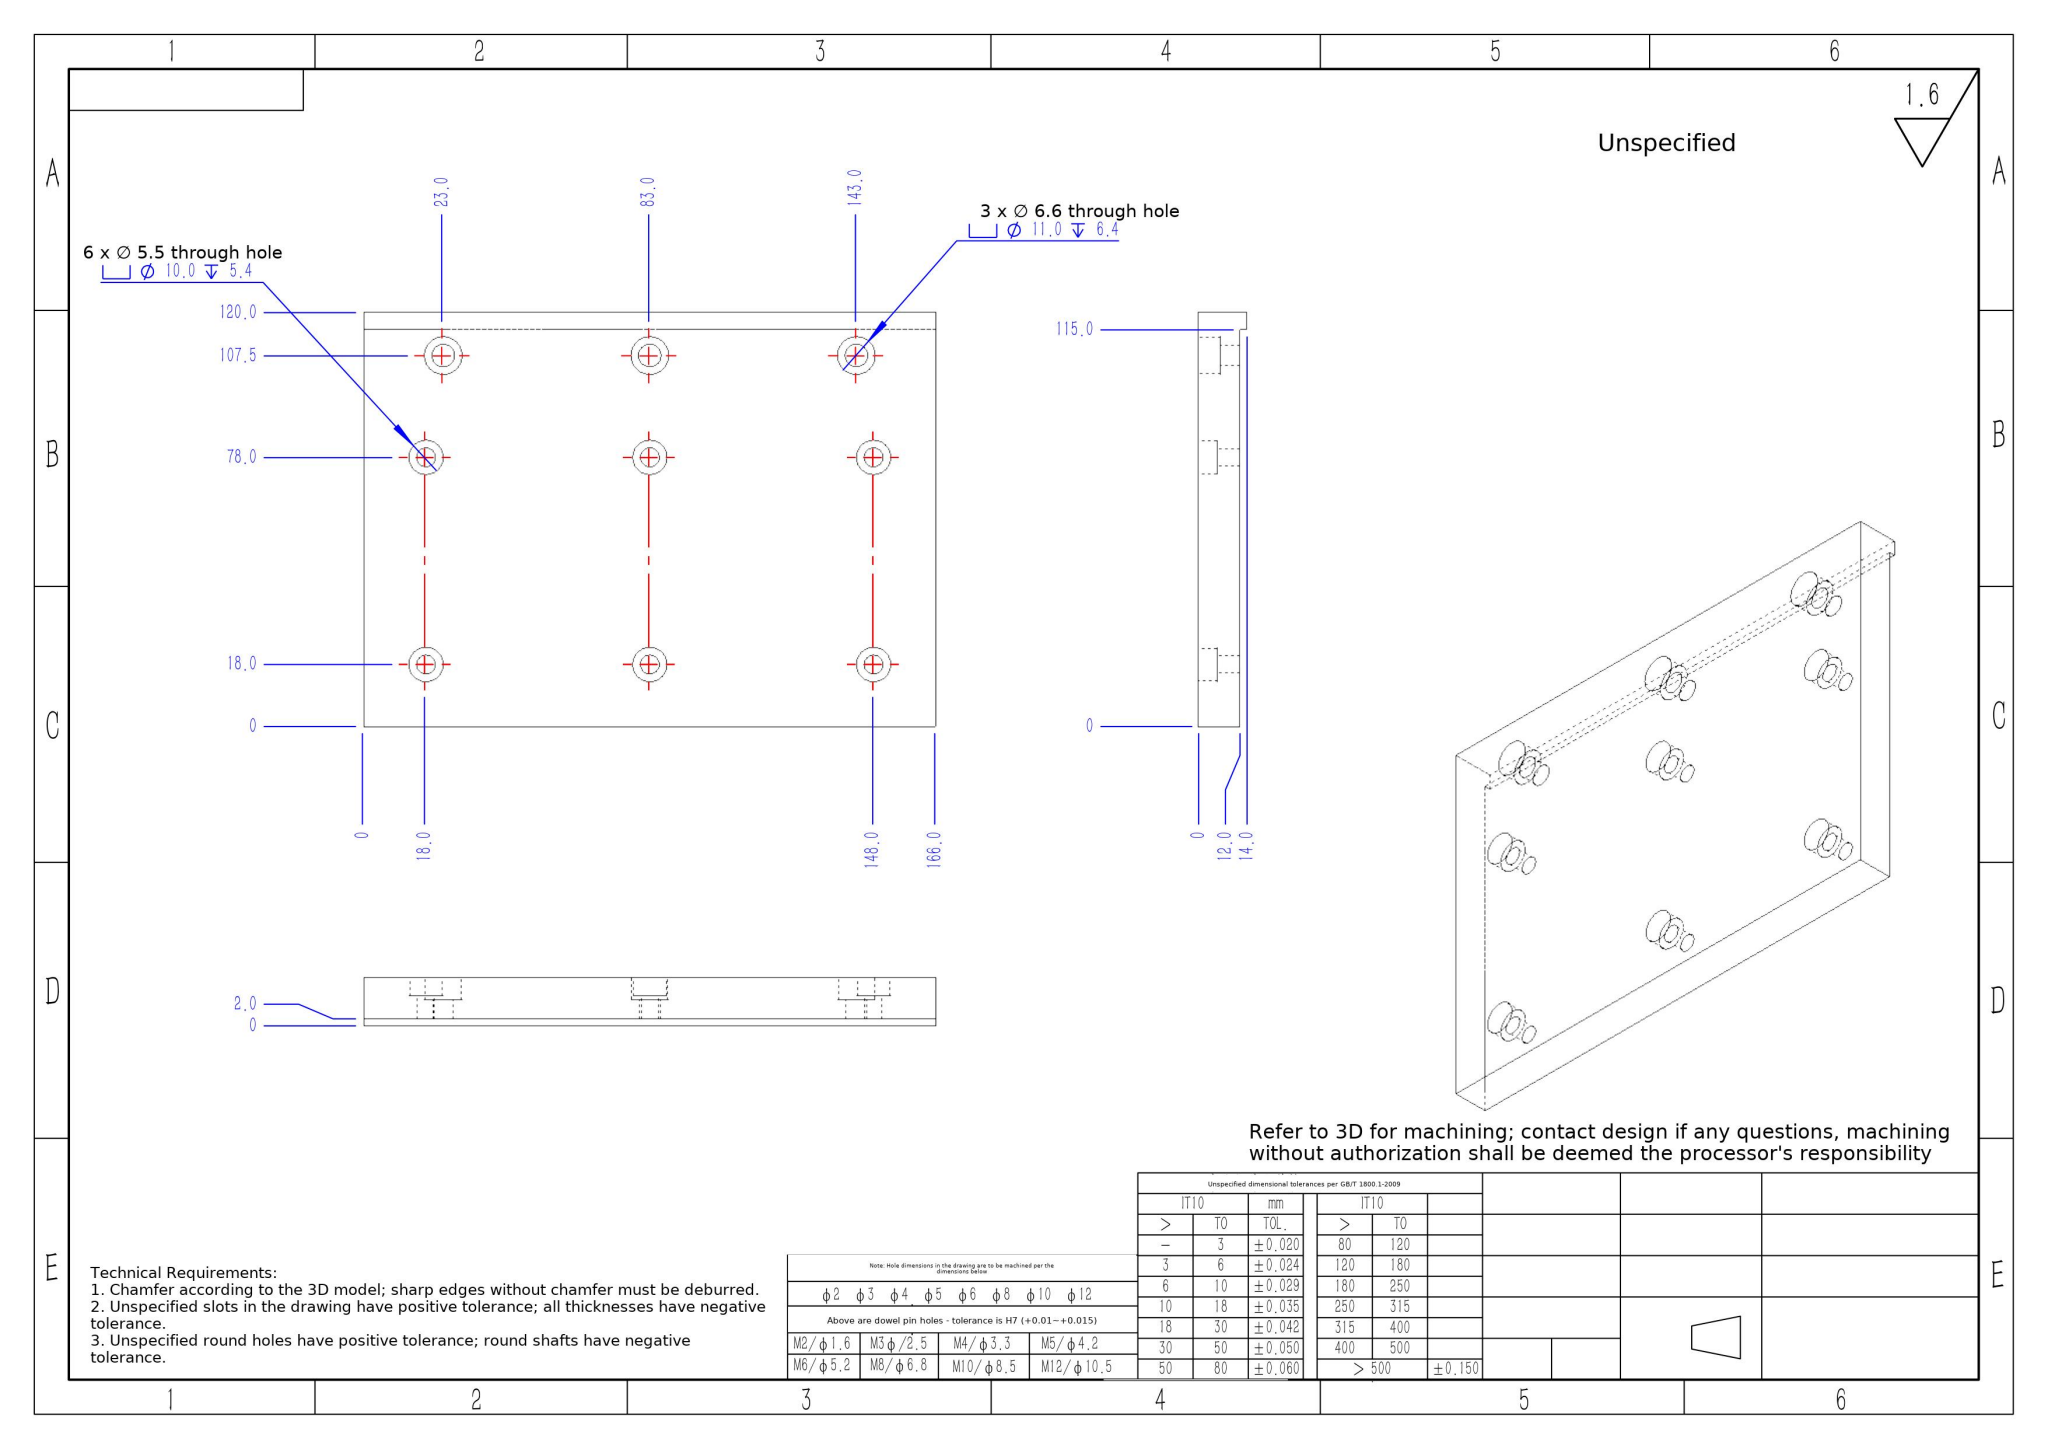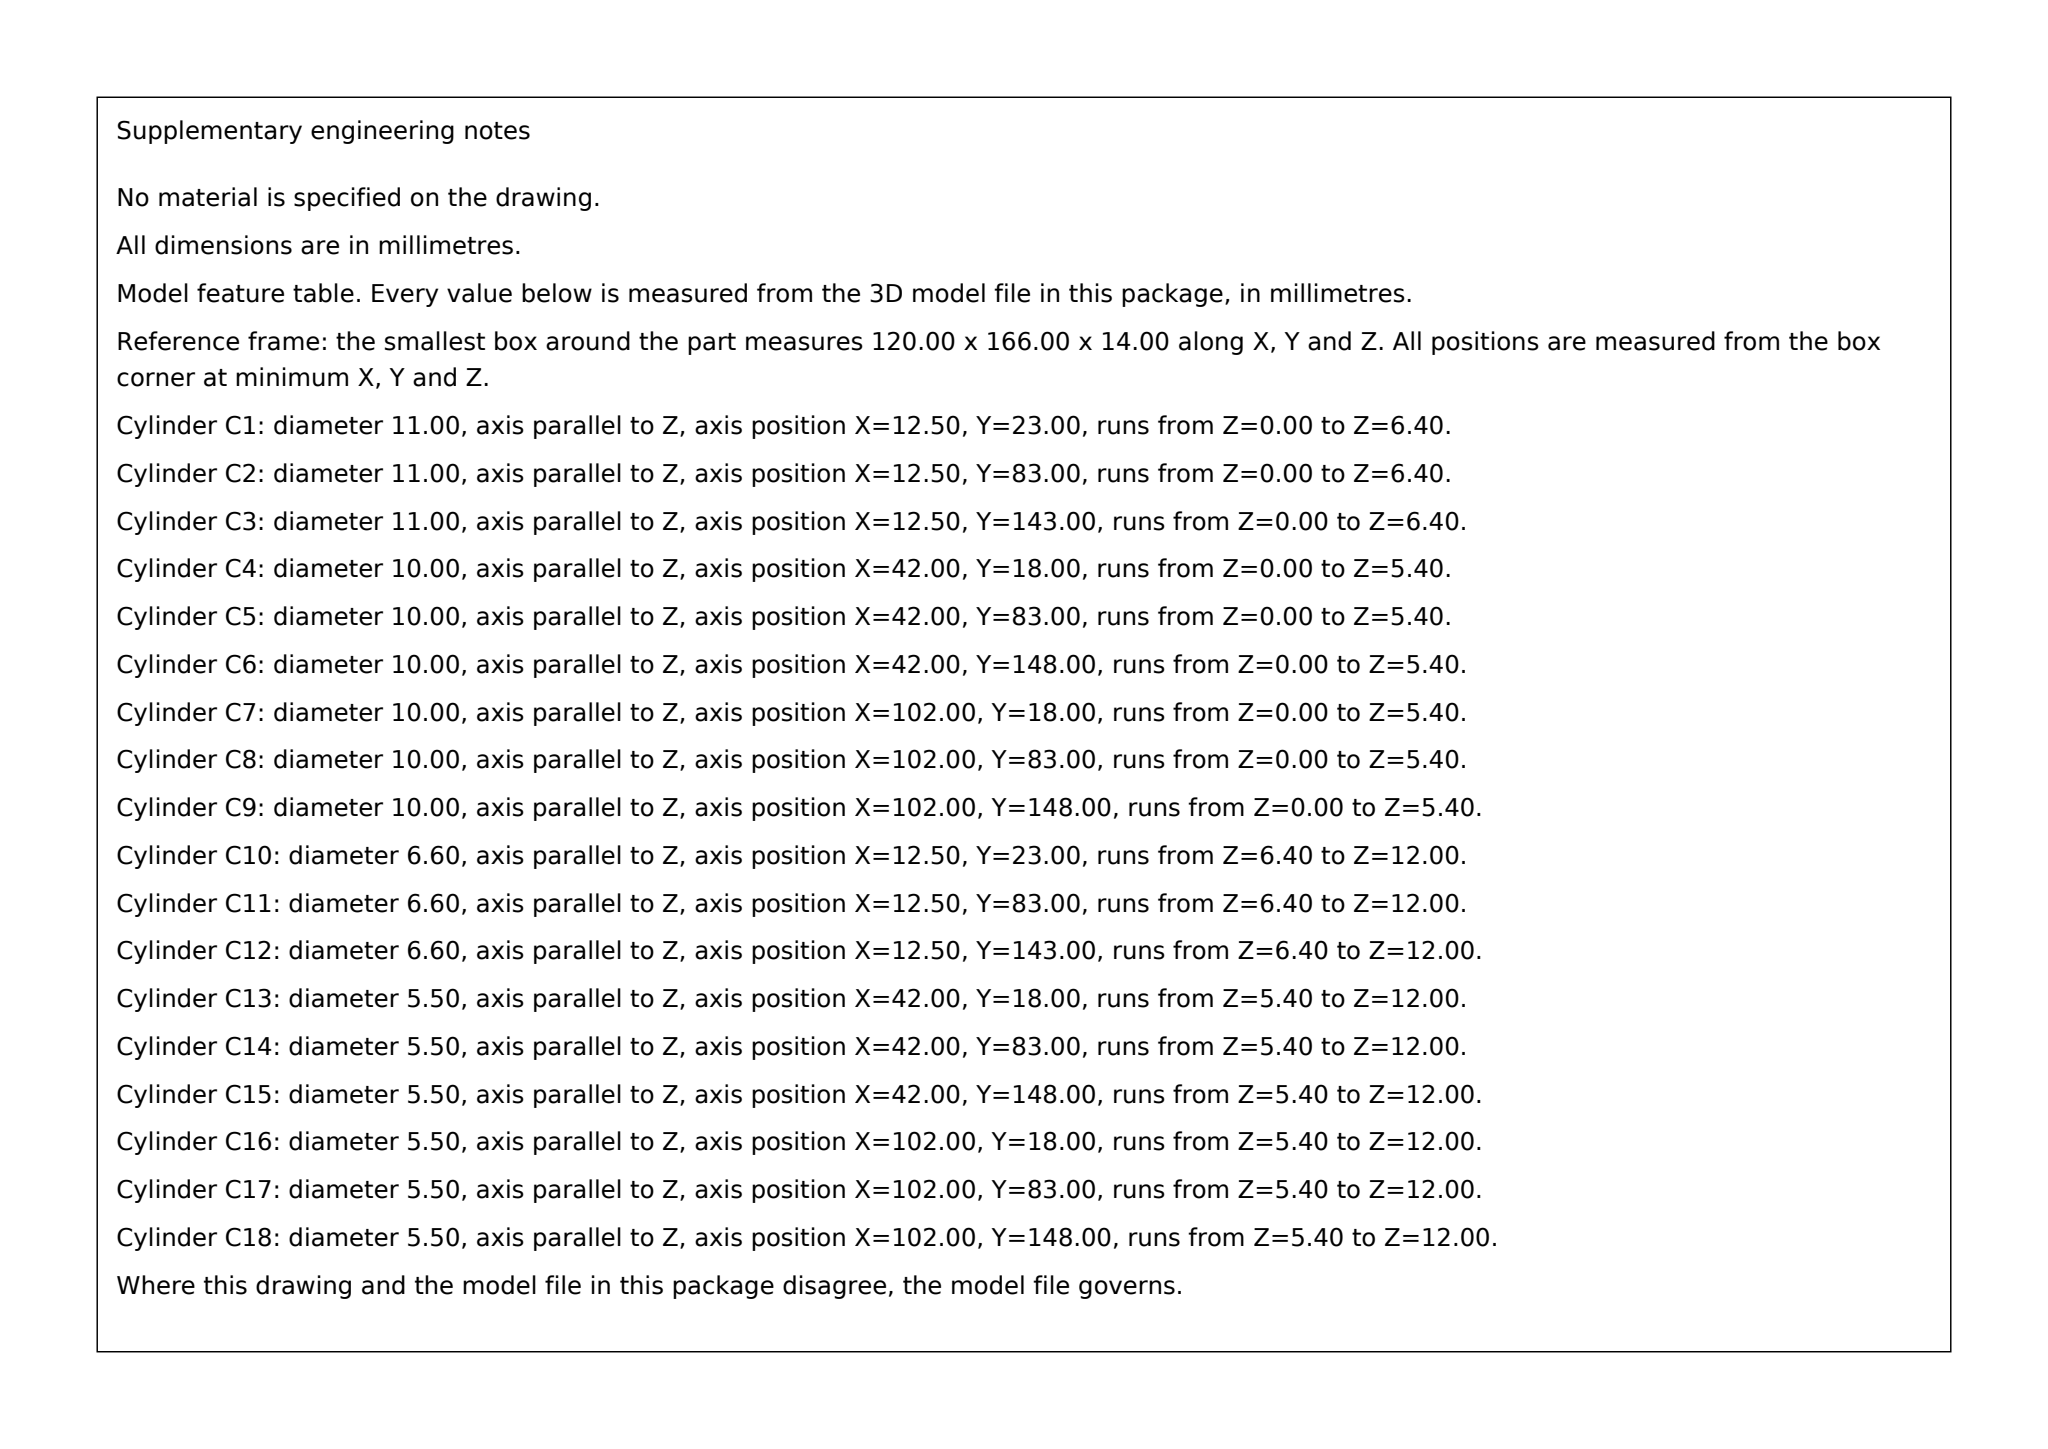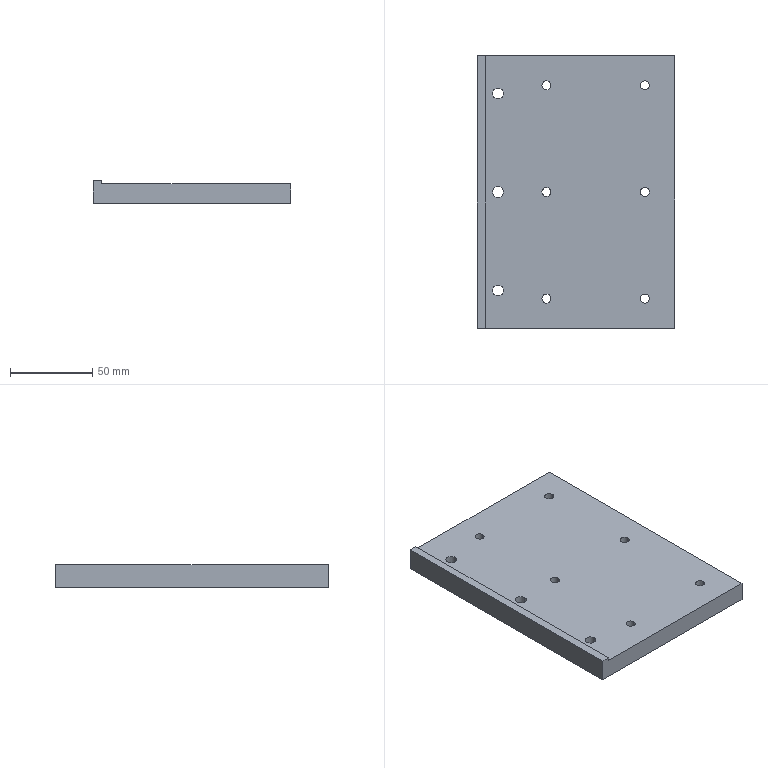Part | SolidWorks | mm | 1 solid | 53 faces | box 120 x 166 x 14 mm | volume 234815 mm3 | cylinder 36 | plane 17 | commonest cylinder face diameters 10 x12 5.5 x12 11 x6 6.6 x6
build123d program:
from build123d import *

# Parameters (mm, degrees)
SKETCH1_W                                       = 120
SKETCH1_H                                       = 166
BOSS_EXTRUDE1_DEPTH                             = 6
SKETCH2_W                                       = 5
SKETCH2_H                                       = 166
BOSS_EXTRUDE2_DEPTH                             = 2
M6_HEX_SOCKET_HEAD_CAP_SCREW_CBORE1_D           = 6.6
M6_HEX_SOCKET_HEAD_CAP_SCREW_CBORE1_DEPTH       = 14
M6_HEX_SOCKET_HEAD_CAP_SCREW_CBORE1_CBORE_D     = 11
M6_HEX_SOCKET_HEAD_CAP_SCREW_CBORE1_CBORE_DEPTH = 6.4
M5_HEX_SOCKET_HEAD_CAP_SCREW_CBORE1_D           = 5.5
M5_HEX_SOCKET_HEAD_CAP_SCREW_CBORE1_CBORE_D     = 10
M5_HEX_SOCKET_HEAD_CAP_SCREW_CBORE1_CBORE_DEPTH = 5.4
LPATTERN1_COUNT                                 = 2
LPATTERN1_PITCH                                 = 60


with BuildPart() as part:
    # Sketch1 → Boss-Extrude1 (new, symmetric)
    with BuildSketch(Plane.XY):
        Rectangle(SKETCH1_W, SKETCH1_H)
    extrude(amount=BOSS_EXTRUDE1_DEPTH, both=True)

    # Sketch2 → Boss-Extrude2 (add)
    with BuildSketch(Plane.XY.offset(6)):
        with Locations((-57.5, 0)):
            Rectangle(SKETCH2_W, SKETCH2_H)
    extrude(amount=BOSS_EXTRUDE2_DEPTH)

    # M6 Hex Socket Head Cap Screw CBORE1
    with Locations(Plane(origin=(0, 0, -6), x_dir=(-1, 0, 0), z_dir=(0, 0, -1))):
        with Locations((47.5, 0), (47.5, 60), (47.5, -60)):
            CounterBoreHole(M6_HEX_SOCKET_HEAD_CAP_SCREW_CBORE1_D / 2, M6_HEX_SOCKET_HEAD_CAP_SCREW_CBORE1_CBORE_D / 2, M6_HEX_SOCKET_HEAD_CAP_SCREW_CBORE1_CBORE_DEPTH, depth=M6_HEX_SOCKET_HEAD_CAP_SCREW_CBORE1_DEPTH)

    # M5 Hex Socket Head Cap Screw CBORE1 (through all)
    with Locations(Plane(origin=(0, 0, -6), x_dir=(-1, 0, 0), z_dir=(0, 0, -1))):
        with Locations((18, -65), (18, 0), (18, 65)):
            m5_hex_socket_head_cap_screw_cbore1 = CounterBoreHole(M5_HEX_SOCKET_HEAD_CAP_SCREW_CBORE1_D / 2, M5_HEX_SOCKET_HEAD_CAP_SCREW_CBORE1_CBORE_D / 2, M5_HEX_SOCKET_HEAD_CAP_SCREW_CBORE1_CBORE_DEPTH)

    # LPattern1: M5 Hex Socket Head Cap Screw CBORE1 ×2
    with Locations(*[(i * LPATTERN1_PITCH, 0, 0) for i in range(1, LPATTERN1_COUNT)]):
        add(m5_hex_socket_head_cap_screw_cbore1, mode=Mode.SUBTRACT)


solid = part.part